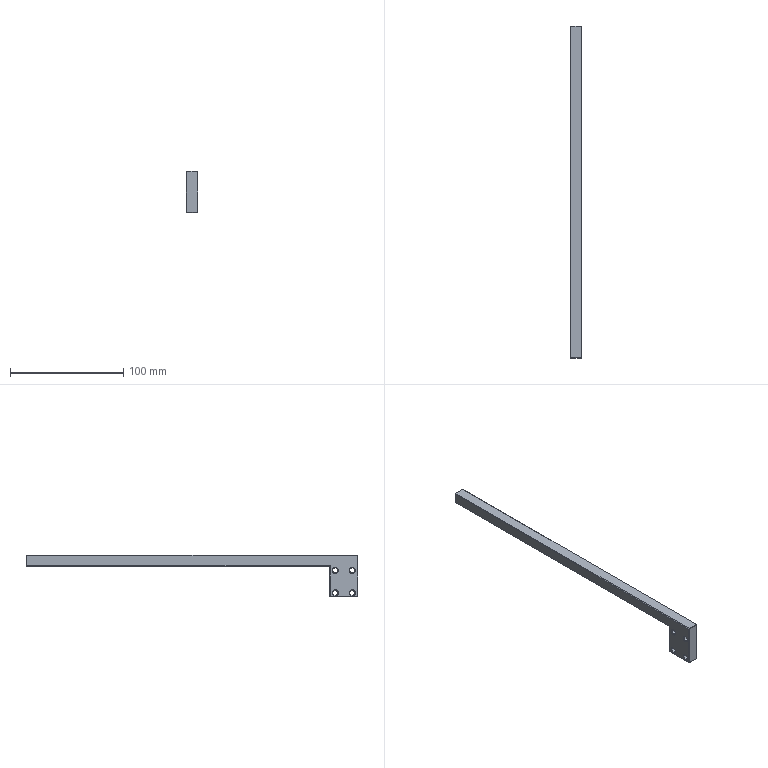Component | SolidWorks | BearingHousingAssembly-1_CylinderJaw2-1 | 1 solid | 60 faces | box 10 x 293 x 37 mm | volume 35107 mm3 | plane 32 | cone 18 | cylinder 10 | commonest cylinder face diameters 4.5 x8 3.3 x2 | material Plain Carbon Steel
build123d program:
from build123d import *

# Parameters (mm, degrees)
BOSS_EXTRUDE1_DEPTH            = 5
F_4_5_4_5_DIAMETER_HOLE1_D     = 4.5
F_4_5_4_5_DIAMETER_HOLE1_DEPTH = 50
F_4_5_4_5_DIAMETER_HOLE1_TIP   = 1.352
CHAMFER1_SIZE                  = 0.5
M4_TAPPED_HOLE1_D              = 3.3
M4_TAPPED_HOLE1_DEPTH          = 14
M4_TAPPED_HOLE1_TIP            = 0.9914


with BuildPart() as part:
    # Sketch1 → Boss-Extrude1 (new, symmetric)
    with BuildSketch(Plane.XY):
        Polygon((0, 0), (0, 293), (10, 293), (10, 25), (37, 25), (37, 0), align=None)
    extrude(amount=BOSS_EXTRUDE1_DEPTH, both=True)

    # 4.5 _4.5_ Diameter Hole1
    with Locations(Plane.XY.offset(5)):
        with Locations((13.5, 20), (33.5, 20), (33.5, 5), (13.5, 5)):
            Hole(F_4_5_4_5_DIAMETER_HOLE1_D / 2, depth=F_4_5_4_5_DIAMETER_HOLE1_DEPTH)
            with Locations((0, 0, -(F_4_5_4_5_DIAMETER_HOLE1_DEPTH + F_4_5_4_5_DIAMETER_HOLE1_TIP / 2))):  # 118° drill point
                Cone(0, F_4_5_4_5_DIAMETER_HOLE1_D / 2, F_4_5_4_5_DIAMETER_HOLE1_TIP, mode=Mode.SUBTRACT)

    # Chamfer1
    chamfer1_edges = [part.edges().sort_by_distance(p)[0] for p in [
        (23.5, 25, 5),
        (0, 0, 0),
        (0, 293, 0),
        (37, 25, 0),
        (37, 0, 0),
        (10, 159, 5),
        (5, 293, 5),
        (0, 146.5, 5),
        (15.75, 5, -5),
        (15.75, 5, 5),
        (35.75, 5, -5),
        (35.75, 5, 5),
        (35.75, 20, -5),
        (35.75, 20, 5),
        (15.75, 20, -5),
        (18.5, 0, 5),
        (15.75, 20, 5),
        (0, 146.5, -5),
        (5, 293, -5),
        (10, 159, -5),
        (37, 12.5, 5),
        (23.5, 25, -5),
        (37, 12.5, -5),
        (18.5, 0, -5),
    ]]
    chamfer(chamfer1_edges, length=CHAMFER1_SIZE)

    # M4 Tapped Hole1
    with Locations(Plane(origin=(0, 293, 0), x_dir=(1, 0, 0), z_dir=(0, 1, 0))):
        with Locations((5, 0)):
            Hole(M4_TAPPED_HOLE1_D / 2, depth=M4_TAPPED_HOLE1_DEPTH)
            with Locations((0, 0, -(M4_TAPPED_HOLE1_DEPTH + M4_TAPPED_HOLE1_TIP / 2))):  # 118° drill point
                Cone(0, M4_TAPPED_HOLE1_D / 2, M4_TAPPED_HOLE1_TIP, mode=Mode.SUBTRACT)


solid = part.part

# Placed as in the assembly
solid = solid.moved(Location((-38.666, 48.064, 4), (0, 90, 0)))